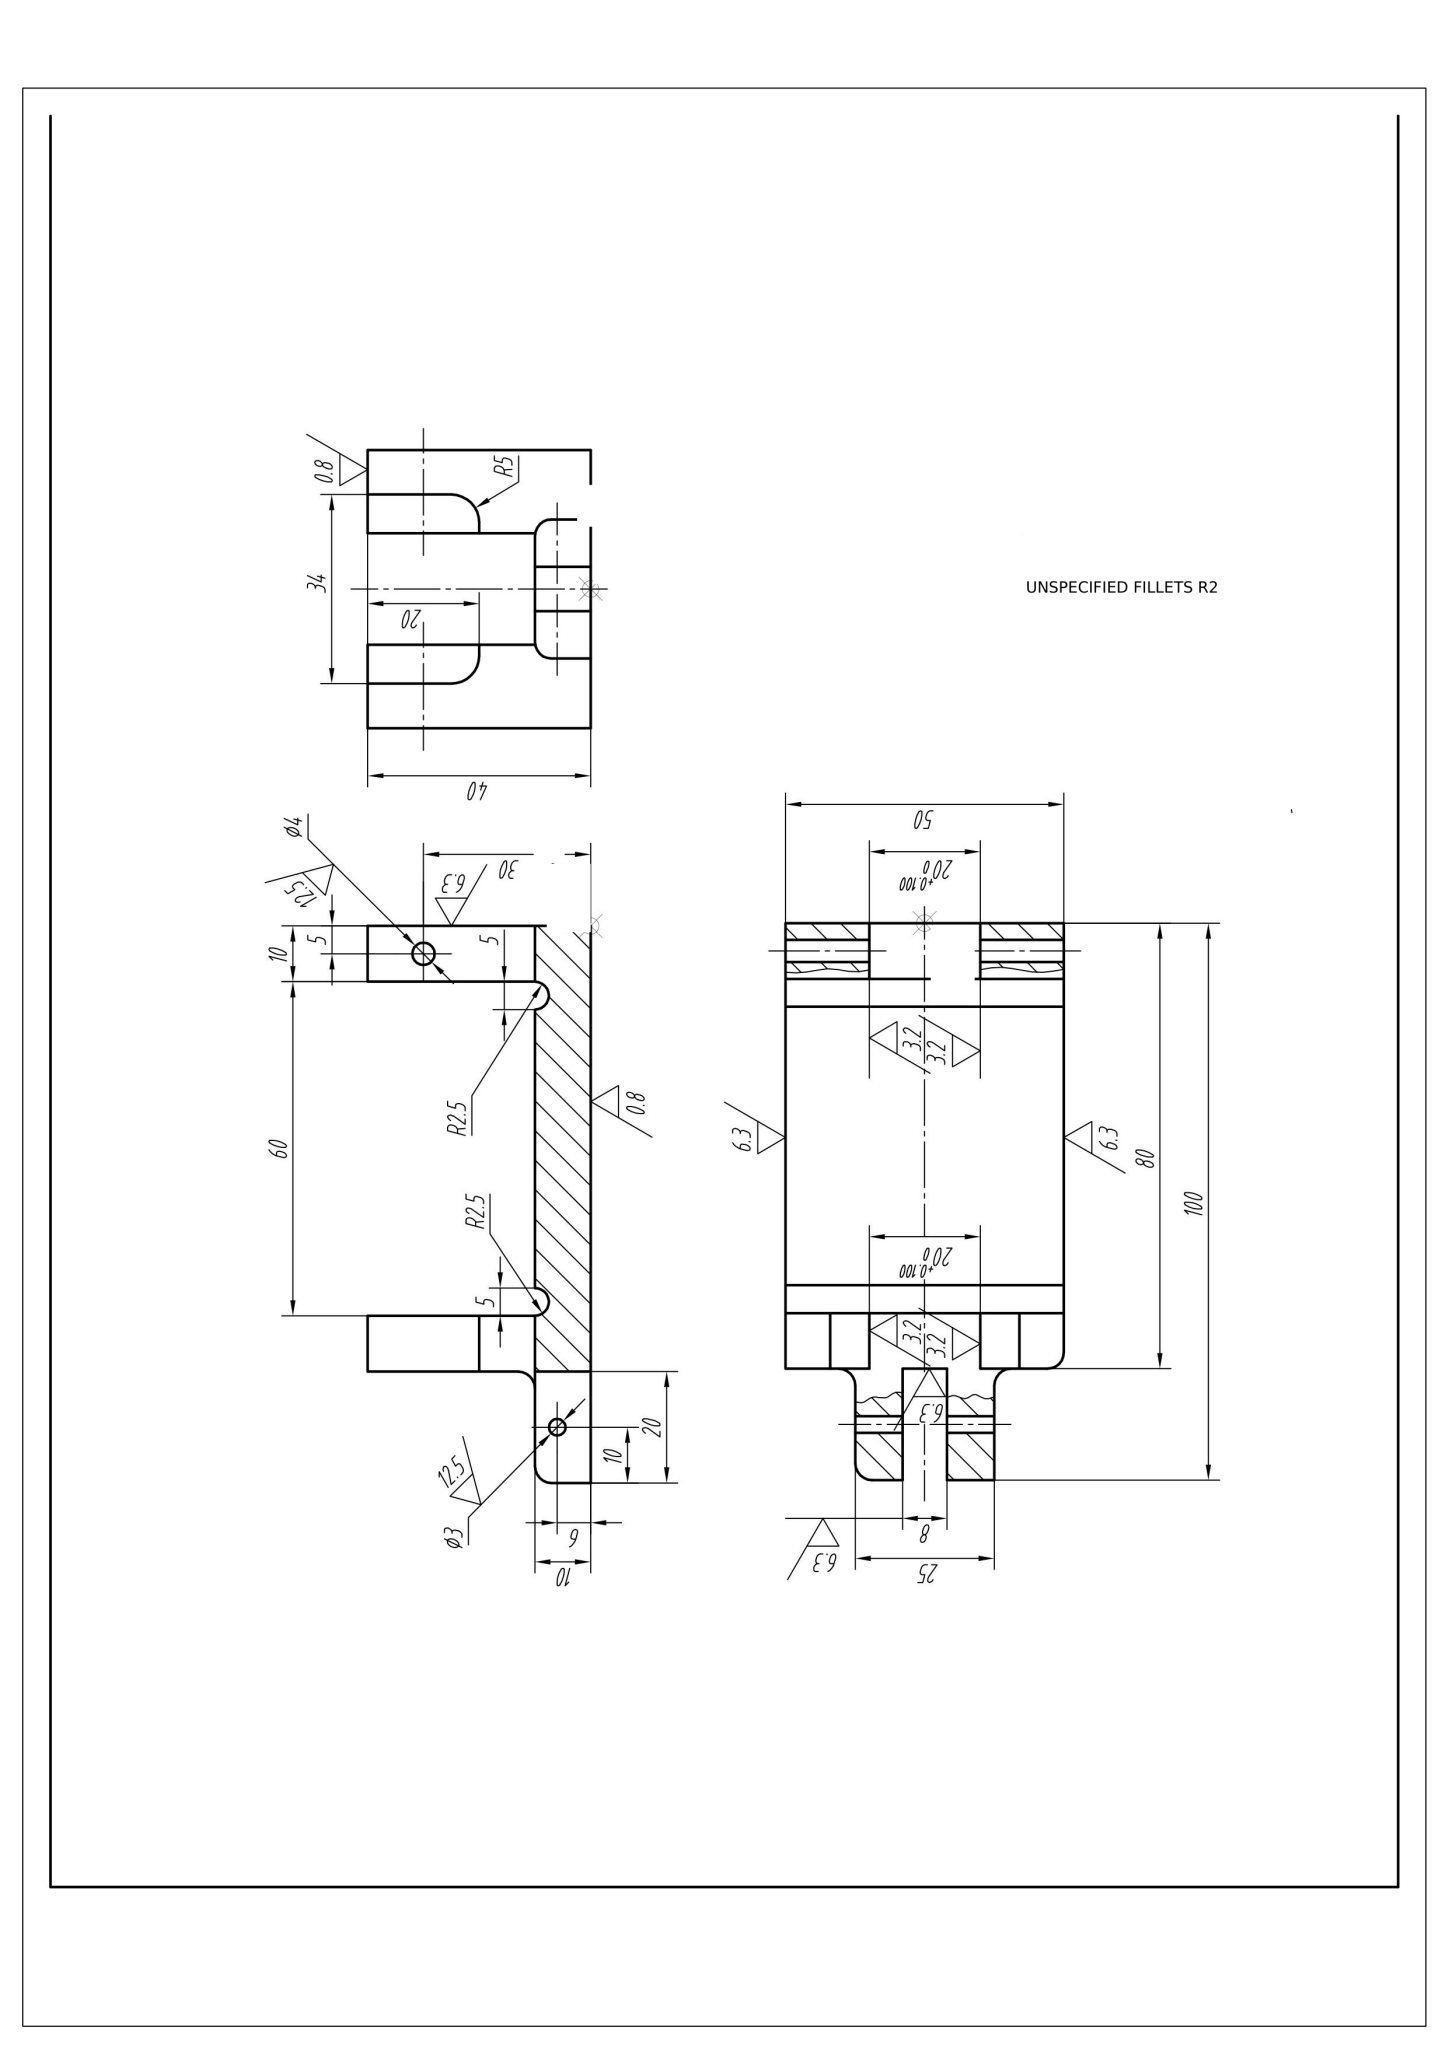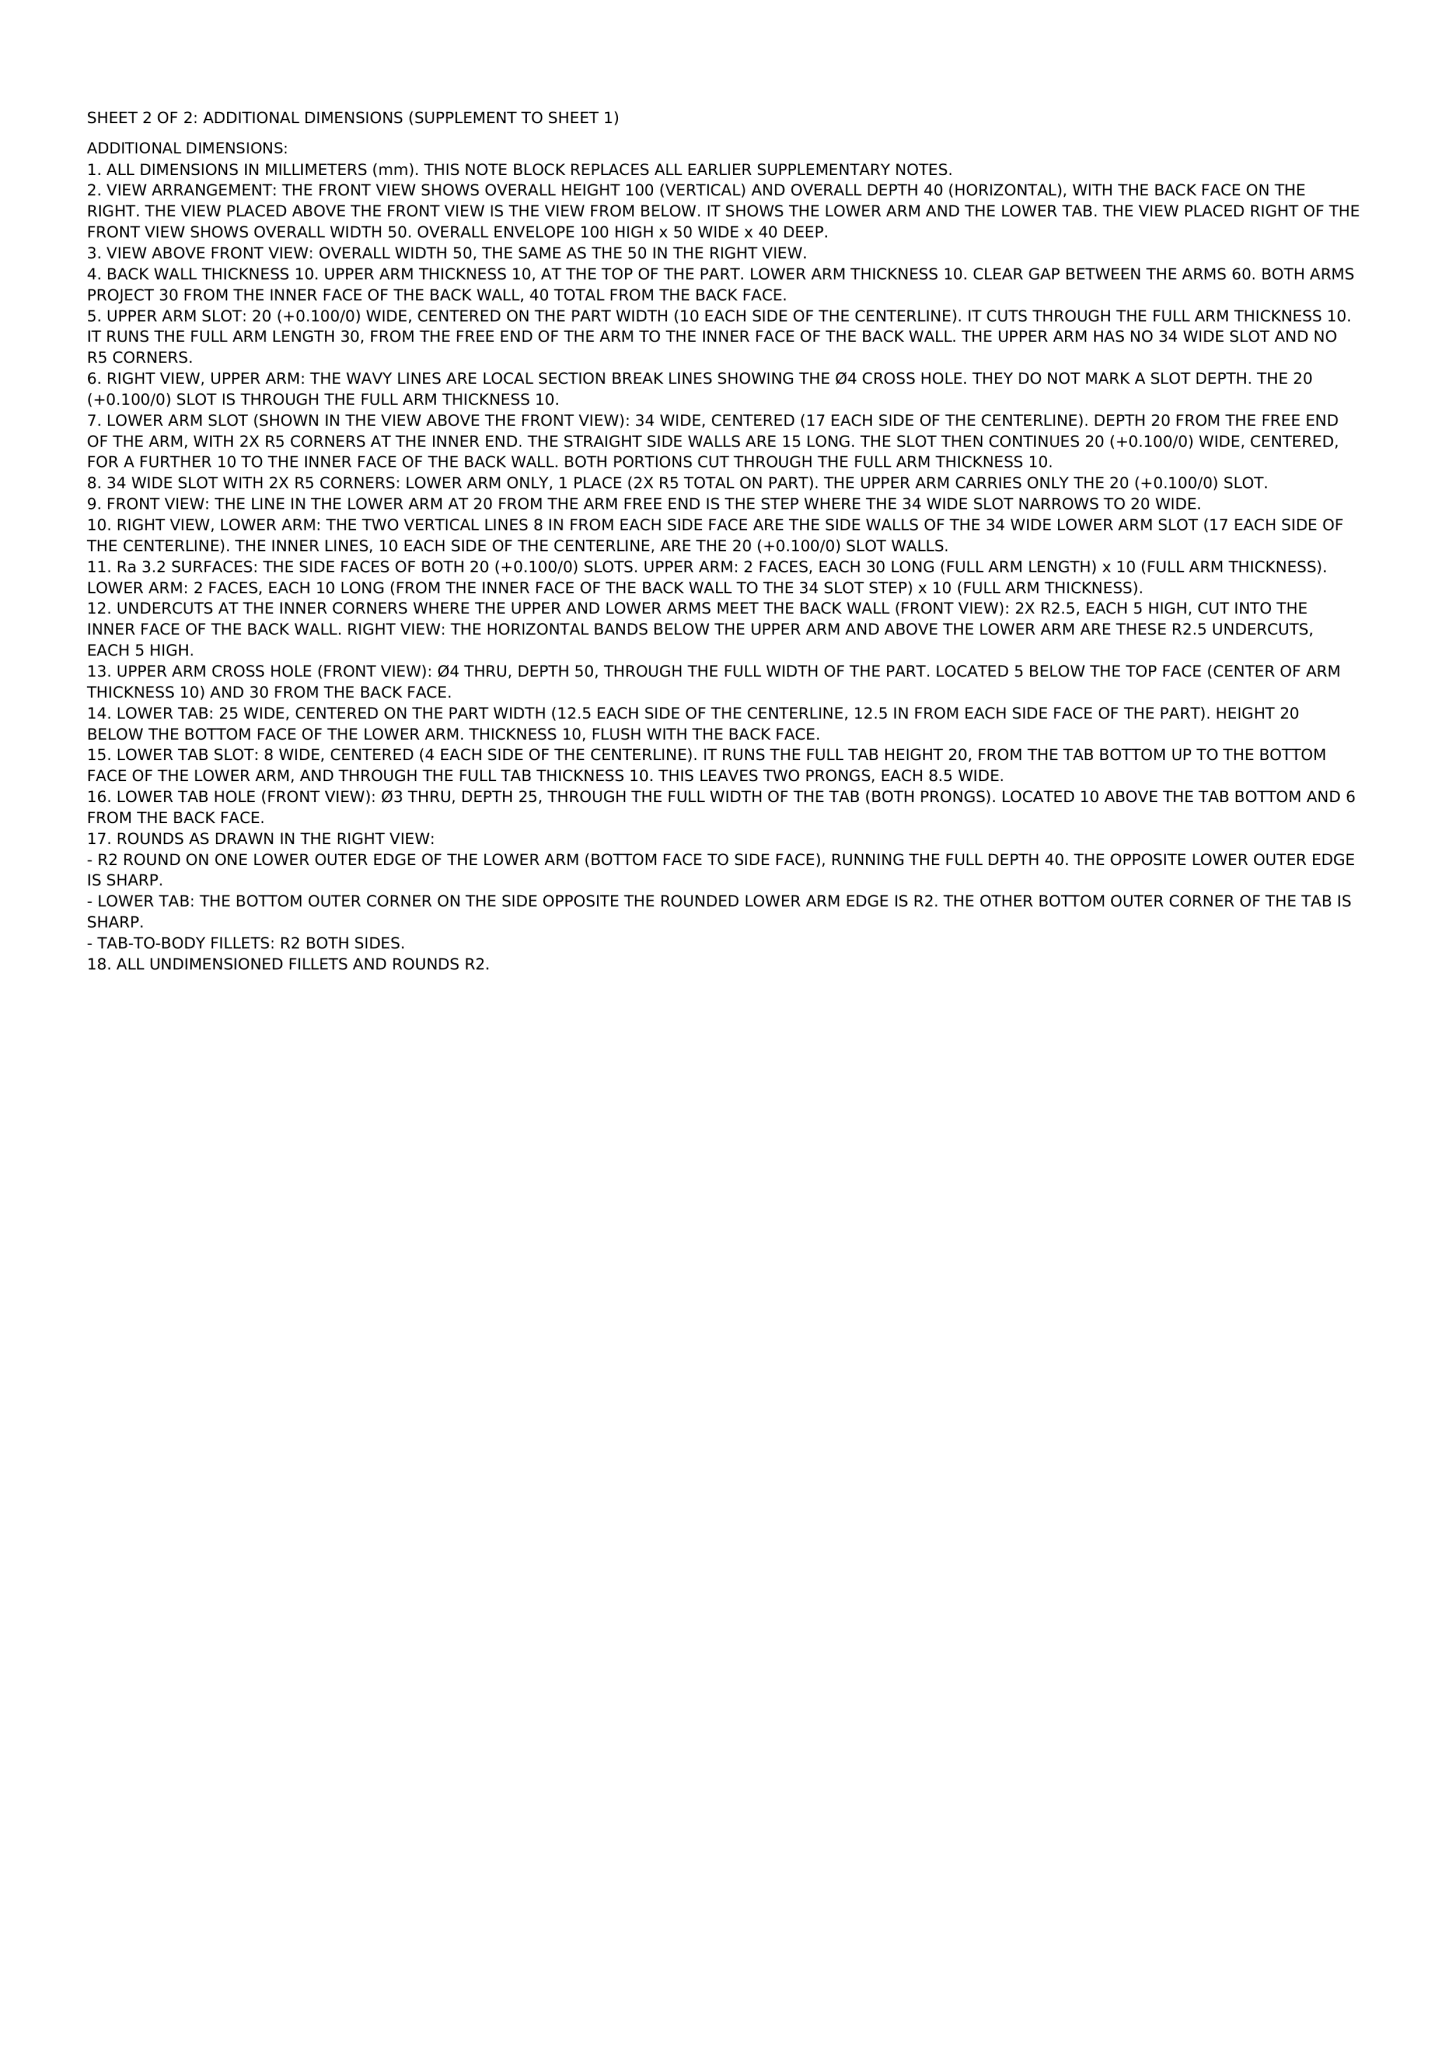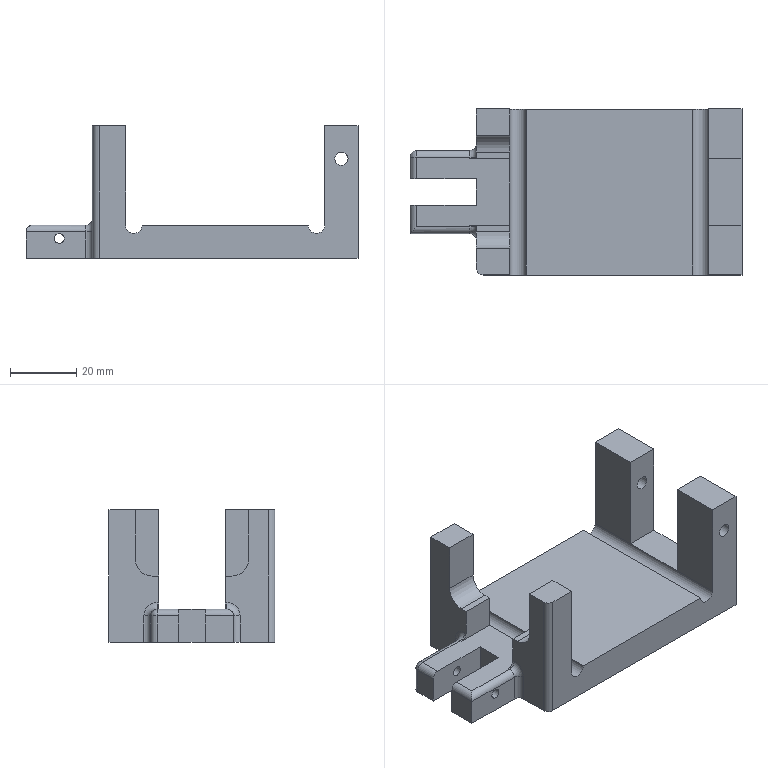Part | NX | mm | 1 solid | 53 faces | box 100 x 50 x 40 mm | volume 57160 mm3 | plane 32 | cylinder 18 | torus 2 | sphere 1 | commonest cylinder face diameters 4 x12 5 x2 10 x2 3 x2